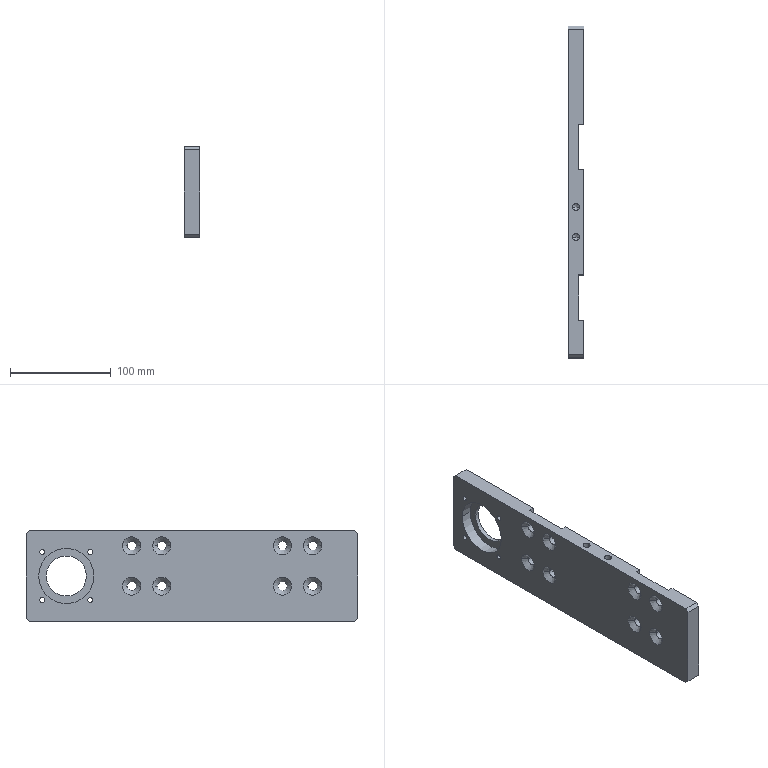Component | SolidWorks | UpperSideBeltXG-XG1-1_UpperSliderConnectingPlateXG-XG1-1 | 1 solid | 71 faces | box 15 x 330 x 90 mm | volume 362825 mm3 | cylinder 32 | cone 20 | plane 19 | commonest cylinder face diameters 9 x16 5 x8 6.8 x4 55 x2 40 x2
build123d program:
from build123d import *

# Parameters (mm, degrees)
SKETCH1_W                                           = 330
SKETCH1_H                                           = 90
BOSS_EXTRUDE1_DEPTH                                 = 7.5
LPATTERN1_COUNT                                     = 2
LPATTERN1_PITCH                                     = 30
LPATTERN1_COUNT_DIR2                                = 2
LPATTERN1_PITCH_DIR2                                = 40
TAPERED_COUNTERSUNK_HOLE_FOR_M8_HEXAGON_D           = 9
TAPERED_COUNTERSUNK_HOLE_FOR_M8_HEXAGON_CSINK_D     = 17.92
TAPERED_COUNTERSUNK_HOLE_FOR_M8_HEXAGON_CSINK_ANGLE = 90
LPATTERN2_COUNT                                     = 2
LPATTERN2_PITCH                                     = 30
LPATTERN2_COUNT_DIR2                                = 2
LPATTERN2_PITCH_DIR2                                = 40
SKETCH6_R                                           = 20
CUT_EXTRUDE1_DEPTH                                  = 15
M6_TAPPED_HOLE1_D                                   = 5
CIRPATTERN1_COUNT                                   = 4
CHAMFER1_SIZE                                       = 3
M8_TAPPED_HOLE1_D                                   = 6.8
M8_TAPPED_HOLE1_DEPTH                               = 19.75
M8_TAPPED_HOLE1_TIP                                 = 2.043
CUT_EXTRUDE2_DEPTH                                  = 189.099
CUT_EXTRUDE2_DEPTH_BACK                             = 189.099
SKETCH12_W                                          = 45
SKETCH12_H                                          = 11.589
SKETCH12_H_2                                        = 12.856
SKETCH13_R                                          = 27.5
CUT_EXTRUDE3_DEPTH                                  = 11


with BuildPart() as part:
    # Sketch1 → Boss-Extrude1 (new, symmetric)
    with BuildSketch(Plane.XY):
        Rectangle(SKETCH1_W, SKETCH1_H)
    extrude(amount=BOSS_EXTRUDE1_DEPTH, both=True)

    # Sketch2 → Countersunk Hole 2 for M8 Hex Socket Cou (revolve, cut)
    with BuildSketch(Plane(origin=(-90, 30, -7.5), x_dir=(0, 1, 0), z_dir=(1, 0, 0))):
        Polygon((0, 0), (0, 24.954), (4.5, 22.25), (4.5, 4.46), (8.96, 0), align=None)
    countersunk_hole_2_for_m8_hex_socket_cou = revolve(axis=Axis((-90, 30, -13.85), (0, 0, 1)), mode=Mode.SUBTRACT)

    # LPattern1: Countersunk Hole 2 for M8 Hex Socket Cou 2 × 2
    with Locations(*[(-i * LPATTERN1_PITCH, -j * LPATTERN1_PITCH_DIR2, 0) for i in range(LPATTERN1_COUNT) for j in range(LPATTERN1_COUNT_DIR2) if (i, j) != (0, 0)]):
        add(countersunk_hole_2_for_m8_hex_socket_cou, mode=Mode.SUBTRACT)

    # Tapered Countersunk Hole for M8 Hexagon (through all)
    with Locations(Plane(origin=(0, 0, -7.5), x_dir=(1, 0, 0), z_dir=(0, 0, -1))):
        with Locations((60, -30)):
            tapered_countersunk_hole_for_m8_hexagon = CounterSinkHole(TAPERED_COUNTERSUNK_HOLE_FOR_M8_HEXAGON_D / 2, TAPERED_COUNTERSUNK_HOLE_FOR_M8_HEXAGON_CSINK_D / 2, counter_sink_angle=TAPERED_COUNTERSUNK_HOLE_FOR_M8_HEXAGON_CSINK_ANGLE)

    # LPattern2: Tapered Countersunk Hole for M8 Hexagon 2 × 2
    with Locations(*[(-i * LPATTERN2_PITCH, -j * LPATTERN2_PITCH_DIR2, 0) for i in range(LPATTERN2_COUNT) for j in range(LPATTERN2_COUNT_DIR2) if (i, j) != (0, 0)]):
        add(tapered_countersunk_hole_for_m8_hexagon, mode=Mode.SUBTRACT)

    # Sketch6 → Cut-Extrude1 (cut)
    with BuildSketch(Plane.XY.offset(7.5)):
        with Locations((125, 0)):
            Circle(SKETCH6_R)
    extrude(amount=-CUT_EXTRUDE1_DEPTH, mode=Mode.SUBTRACT)

    # M6 Tapped Hole1 (through all)
    with Locations(Plane.XY.offset(7.5)):
        with Locations((101.135, 23.865)):
            m6_tapped_hole1 = Hole(M6_TAPPED_HOLE1_D / 2)

    # CirPattern1: M6 Tapped Hole1 ×4 about axis
    cirpattern1_axis = Axis((125, 0, 0), (0, 0, 1))
    for i in range(1, CIRPATTERN1_COUNT):
        add(m6_tapped_hole1.rotate(cirpattern1_axis, i * 360 / CIRPATTERN1_COUNT), mode=Mode.SUBTRACT)

    # Chamfer1
    chamfer1_edges = [part.edges().sort_by_distance(p)[0] for p in [
        (165, -45, 0),
        (-165, -45, 0),
        (-165, 45, 0),
        (165, 45, 0),
    ]]
    chamfer(chamfer1_edges, length=CHAMFER1_SIZE)

    # M8 Tapped Hole1
    with Locations(Plane(origin=(0, 45, 0), x_dir=(1, 0, 0), z_dir=(0, 1, 0))):
        with Locations((-45, 0), (-15, 0)):
            Hole(M8_TAPPED_HOLE1_D / 2, depth=M8_TAPPED_HOLE1_DEPTH)
            with Locations((0, 0, -(M8_TAPPED_HOLE1_DEPTH + M8_TAPPED_HOLE1_TIP / 2))):  # 118° drill point
                Cone(0, M8_TAPPED_HOLE1_D / 2, M8_TAPPED_HOLE1_TIP, mode=Mode.SUBTRACT)

    # Sketch12 → Cut-Extrude2 (cut, two sides: drawn at the far end of the back side and taken through both)
    with BuildSketch(Plane(origin=(0, 45, 0), x_dir=(1, 0, 0), z_dir=(0, 1, 0)).offset(-CUT_EXTRUDE2_DEPTH_BACK)):
        with Locations((-105, -8.294)):
            Rectangle(SKETCH12_W, SKETCH12_H)
        with Locations((45, -8.928)):
            Rectangle(SKETCH12_W, SKETCH12_H_2)
    extrude(amount=CUT_EXTRUDE2_DEPTH + CUT_EXTRUDE2_DEPTH_BACK, mode=Mode.SUBTRACT)

    # Sketch13 → Cut-Extrude3 (cut)
    with BuildSketch(Plane(origin=(0, 0, -7.5), x_dir=(-1, 0, 0), z_dir=(0, 0, -1))):
        with Locations((-125, 0)):
            Circle(SKETCH13_R)
    extrude(amount=-CUT_EXTRUDE3_DEPTH, mode=Mode.SUBTRACT)


solid = part.part

# Placed as in the assembly
solid = solid.moved(Location((-373.72, 500, 263), (90, 90, 0)))